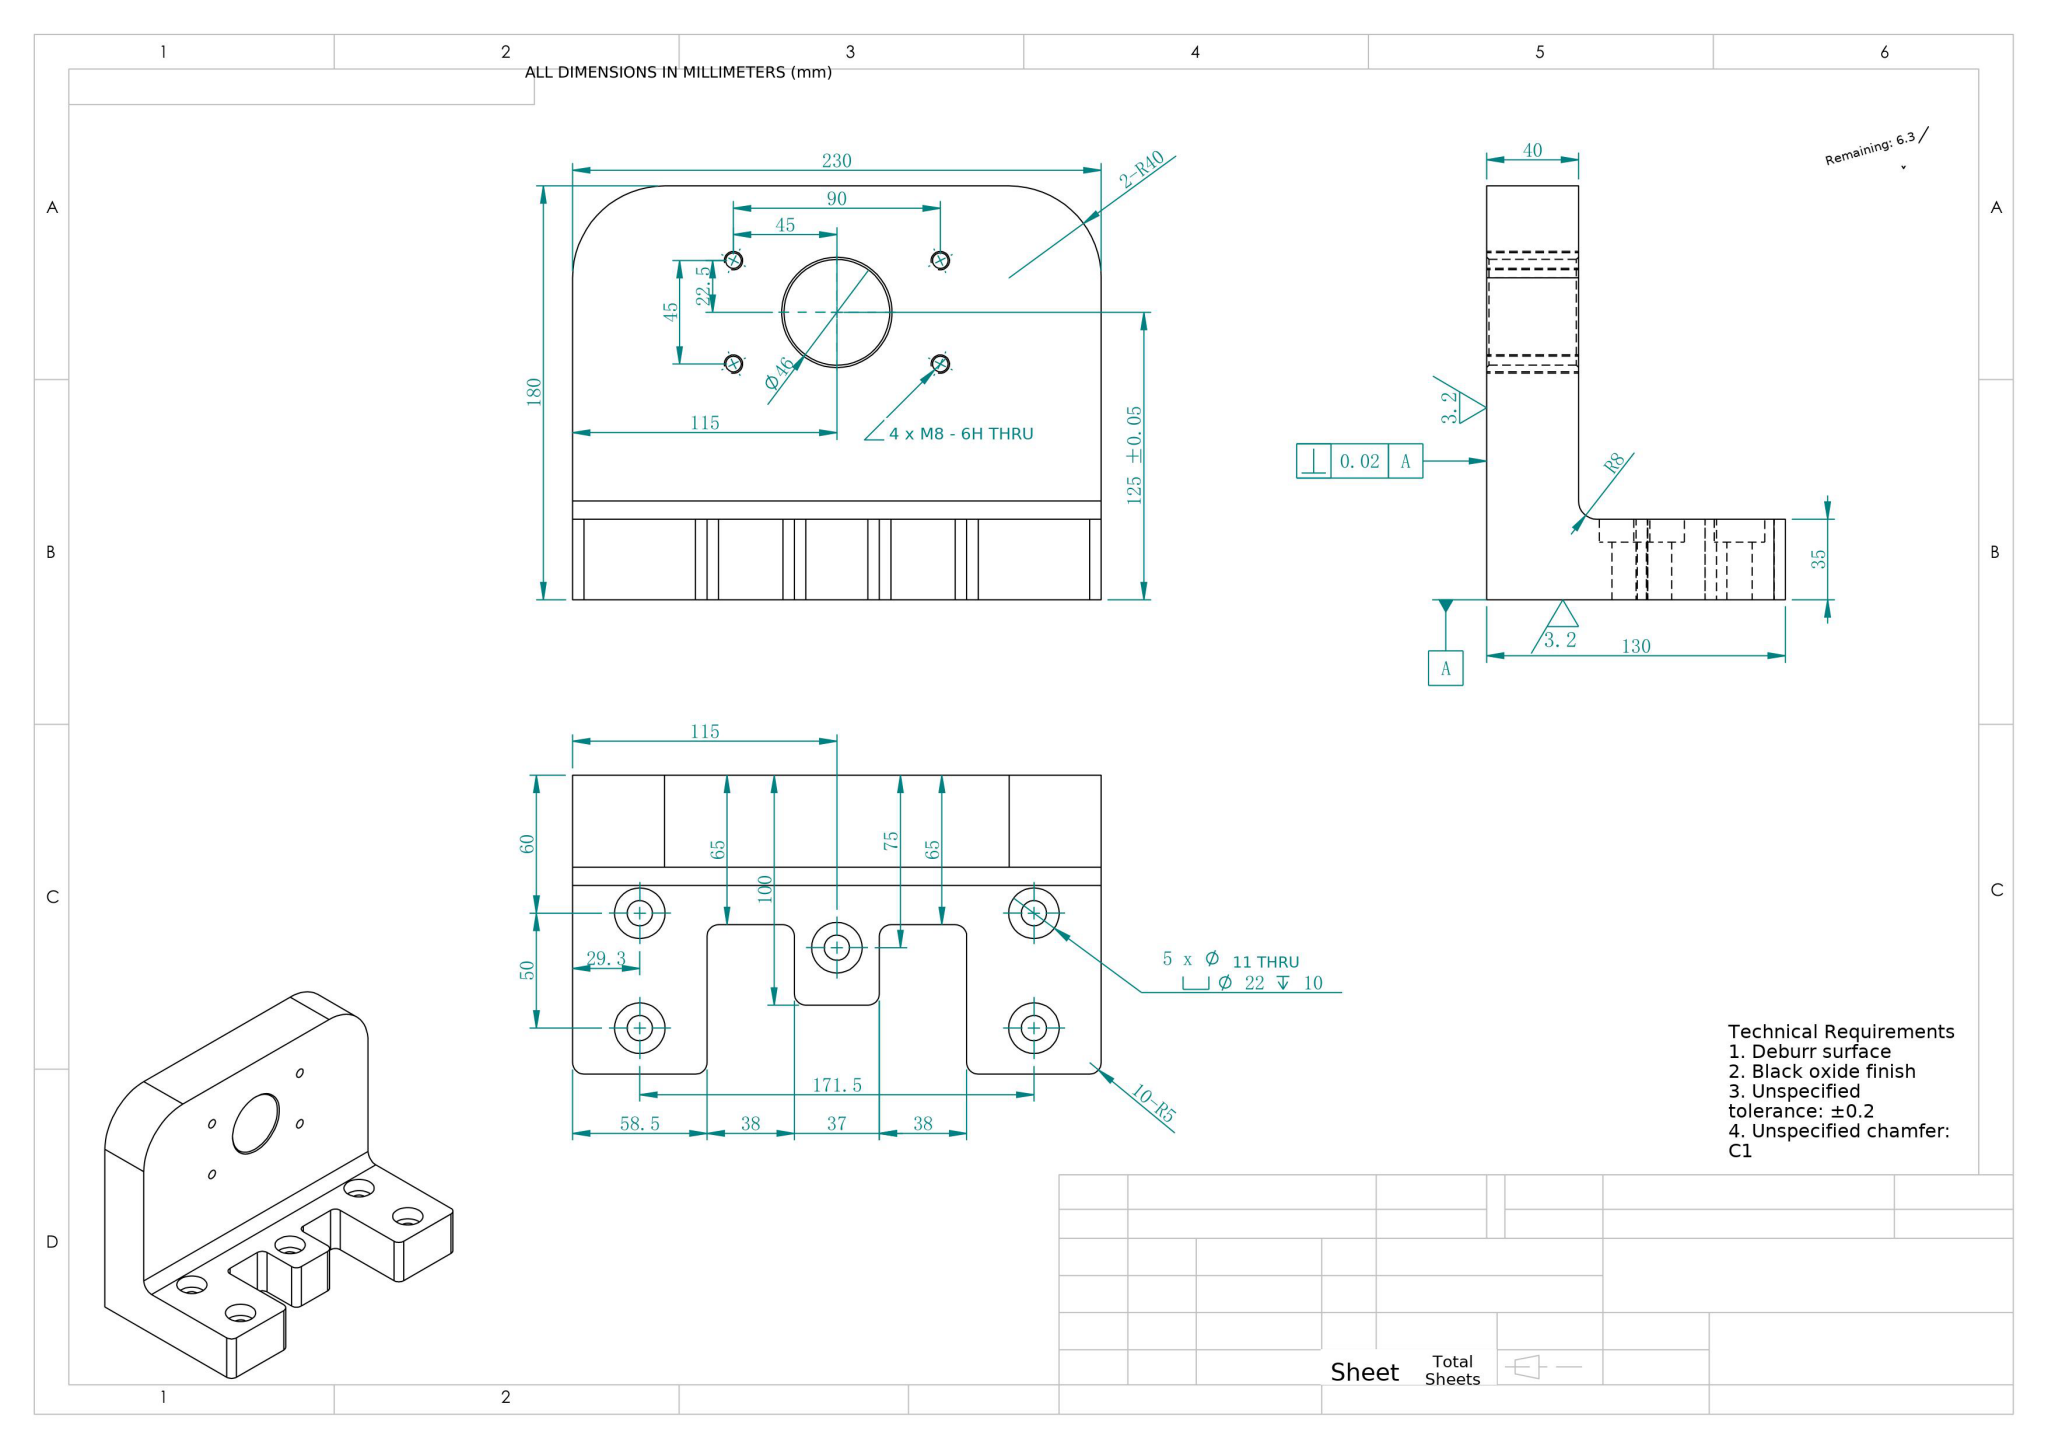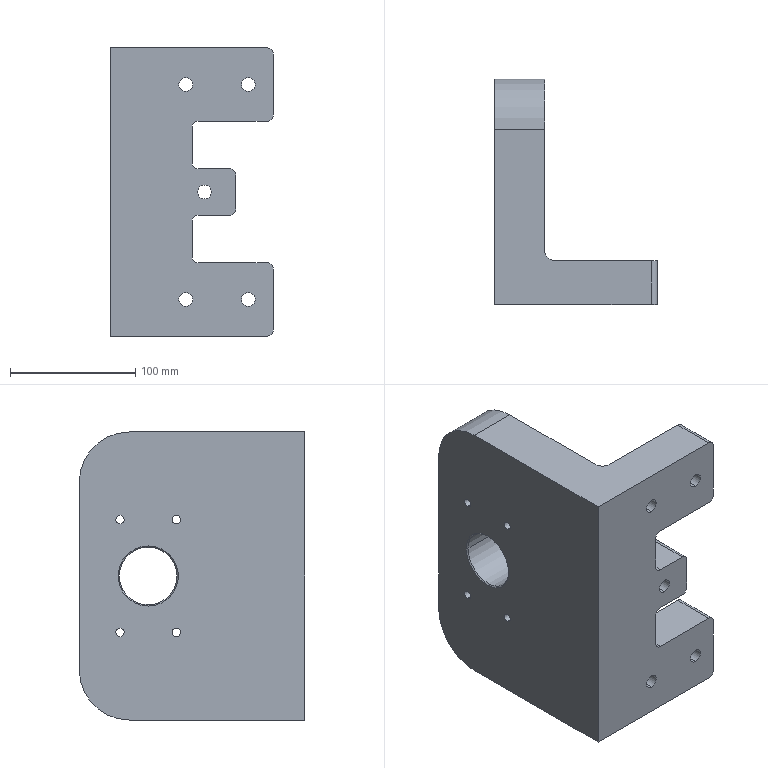Part | NX | mm | 1 solid | 68 faces | box 130 x 180 x 230 mm | volume 2040745 mm3 | cylinder 43 | plane 21 | cone 4 | commonest cylinder face diameters 22 x10 11 x10 10 x10 6.8 x8 46 x2 80 x2 16 x1